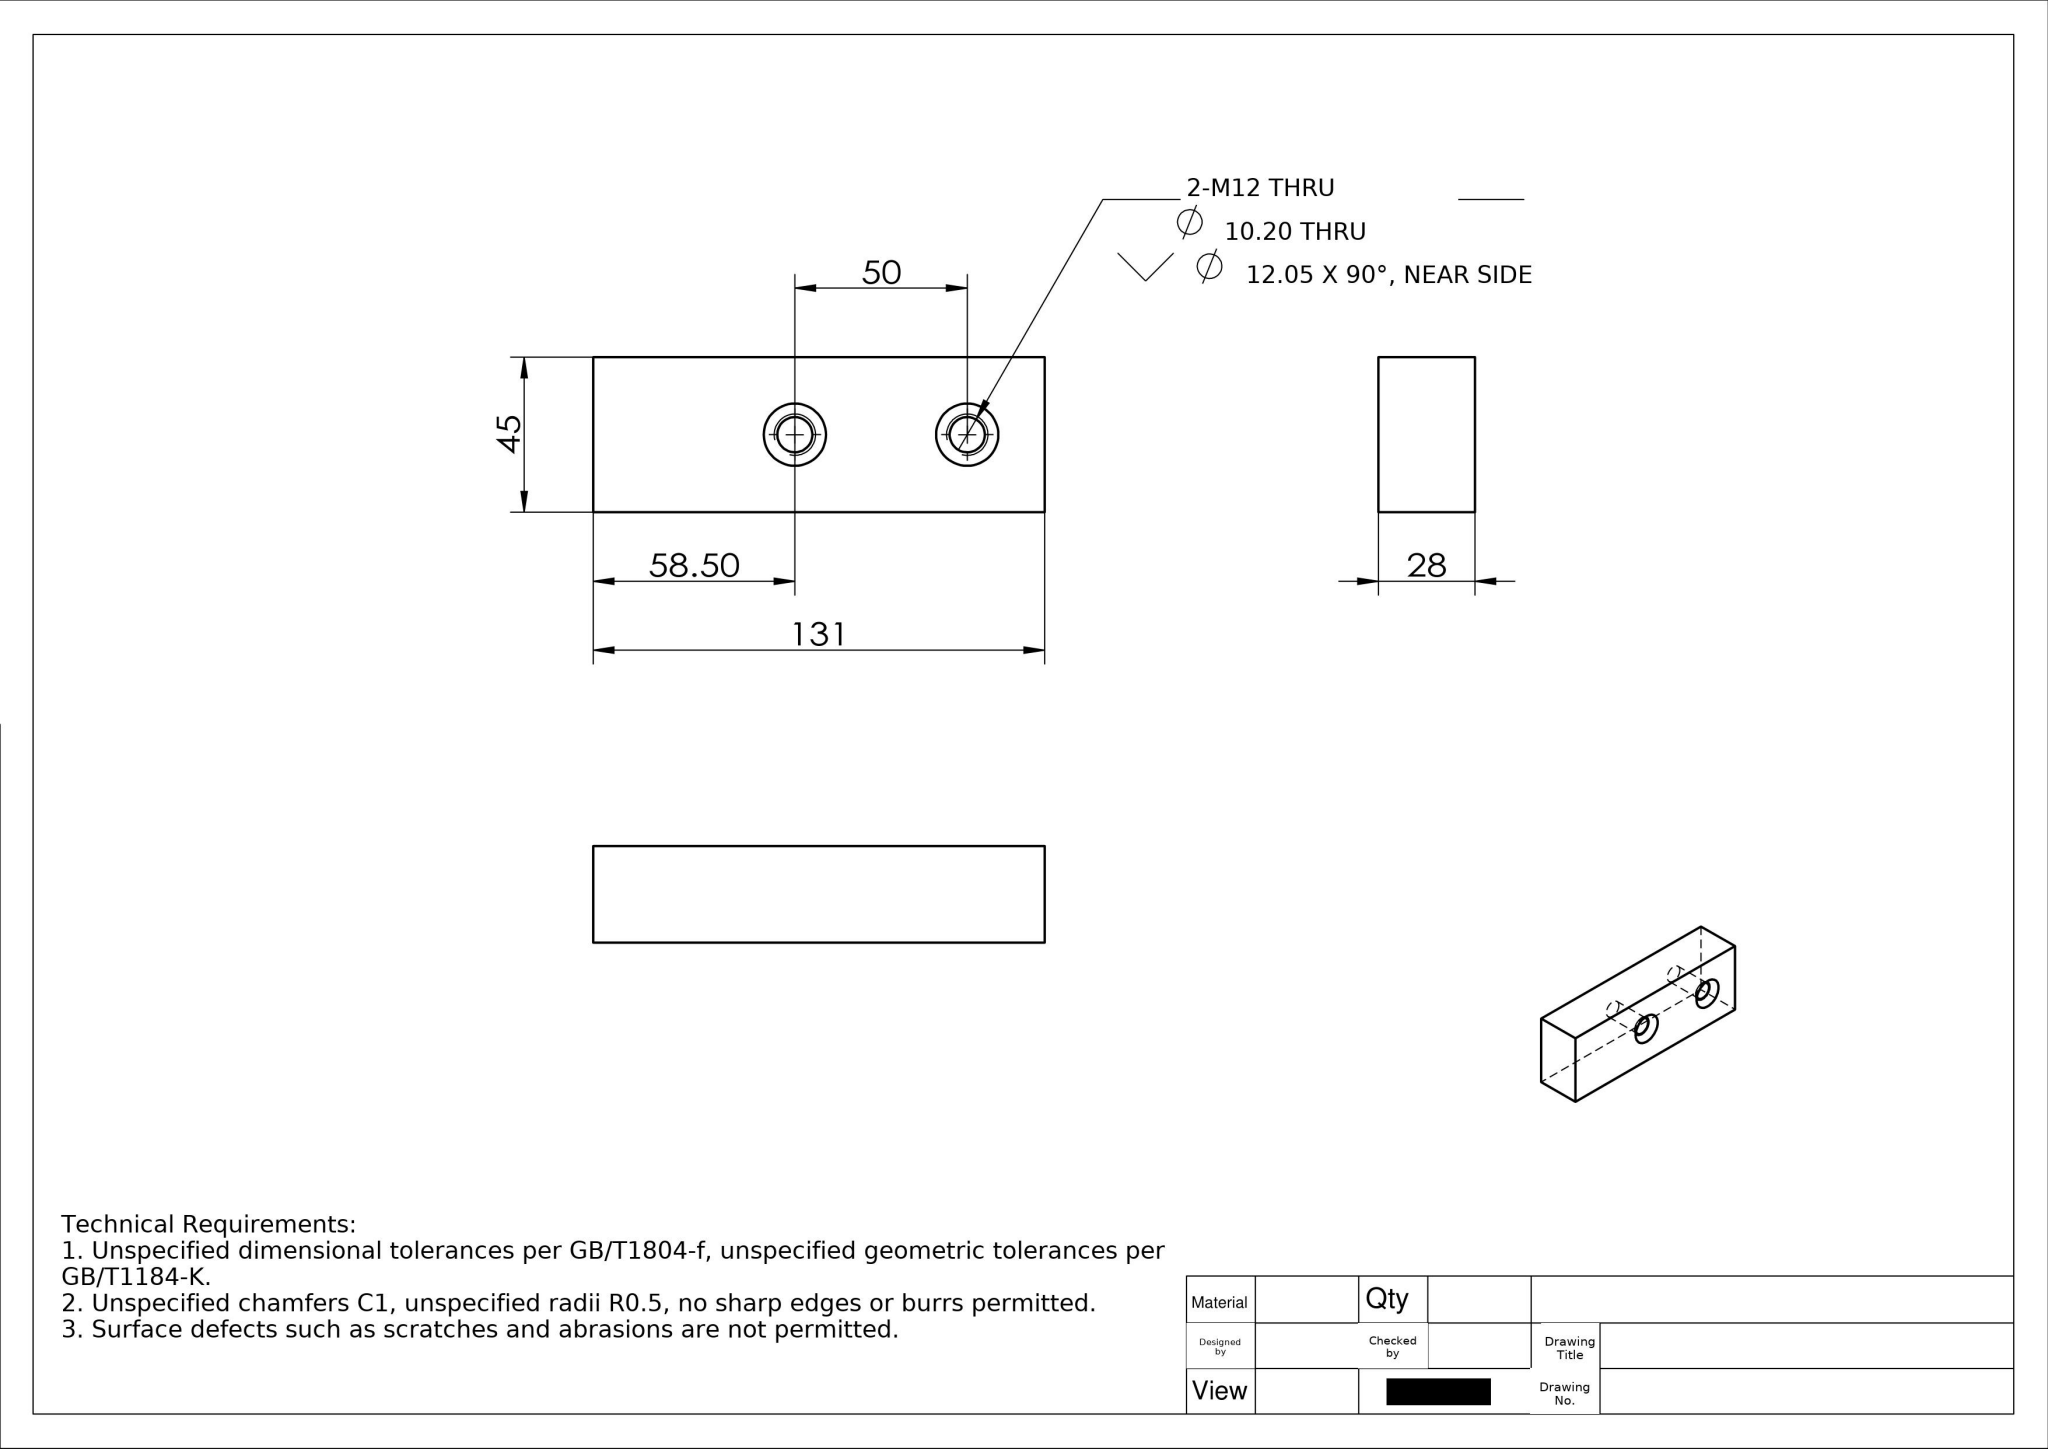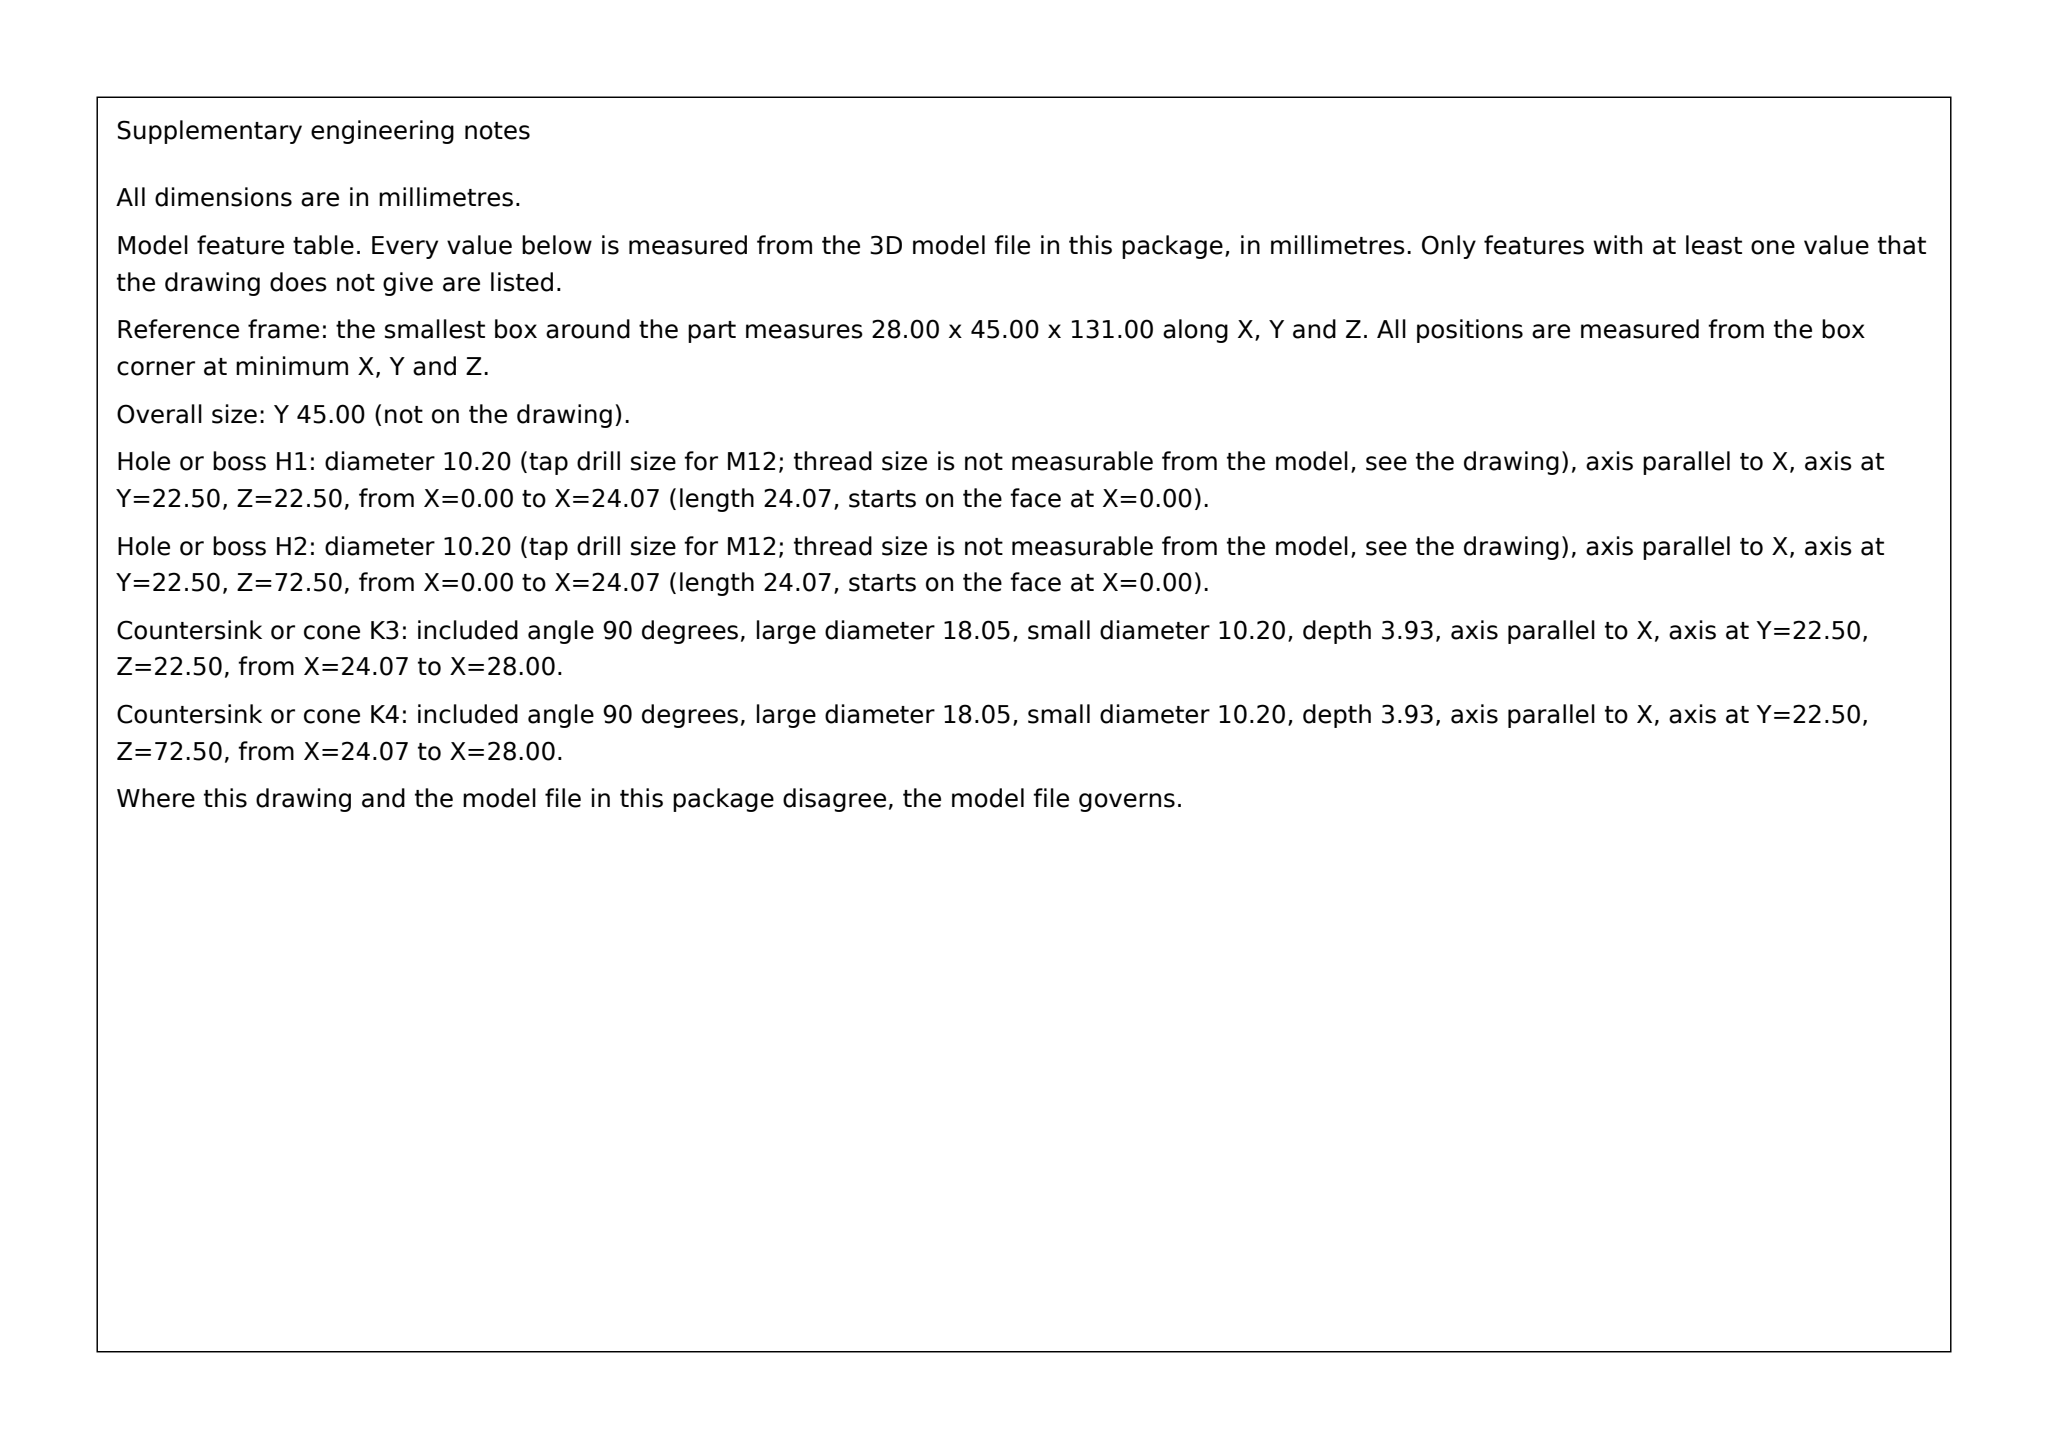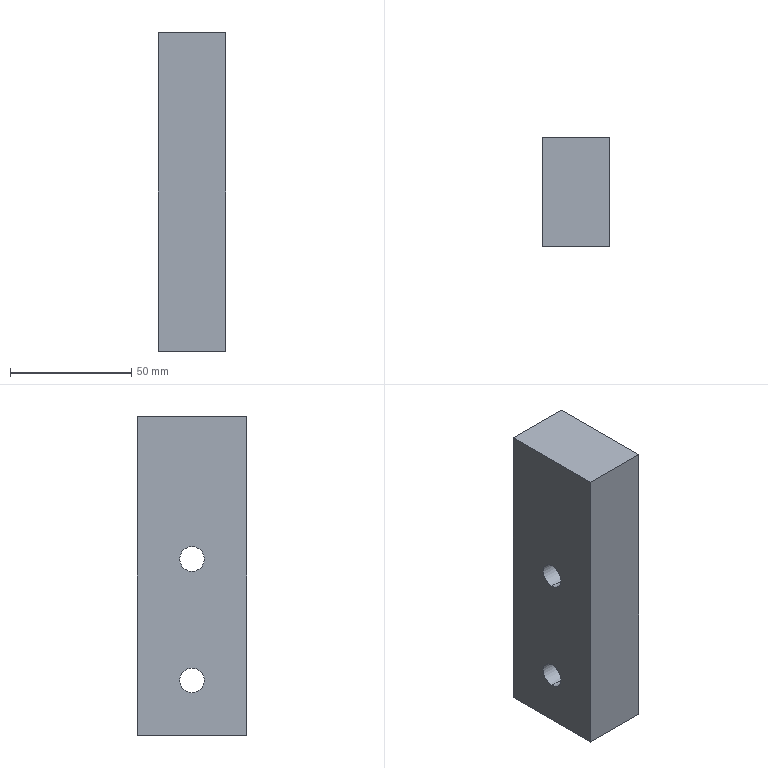Part | SolidWorks | mm | 1 solid | 14 faces | box 28 x 45 x 131 mm | volume 159864 mm3 | plane 6 | cone 4 | cylinder 4 | commonest cylinder face diameters 10.2 x4
STEP:
#1=CARTESIAN_POINT('',(-0.925,22.5,77.6));
#2=VERTEX_POINT('',#1);
#3=CARTESIAN_POINT('',(-0.925,22.5,67.4));
#4=VERTEX_POINT('',#3);
#5=CARTESIAN_POINT('',(-0.925,22.5,72.5));
#6=DIRECTION('',(1.,0.,0.));
#7=DIRECTION('',(0.,0.,-1.));
#8=AXIS2_PLACEMENT_3D('',#5,#6,#7);
#9=CIRCLE('',#8,5.1);
#10=EDGE_CURVE('',#2,#4,#9,.T.);
#11=ORIENTED_EDGE('',*,*,#10,.F.);
#12=CARTESIAN_POINT('',(3.,22.5,81.525));
#13=VERTEX_POINT('',#12);
#14=CARTESIAN_POINT('',(0.,22.5,78.525));
#15=DIRECTION('',(0.7071,0.,0.7071));
#16=VECTOR('',#15,1000.);
#17=LINE('',#14,#16);
#18=EDGE_CURVE('',#2,#13,#17,.T.);
#19=ORIENTED_EDGE('',*,*,#18,.T.);
#20=CARTESIAN_POINT('',(3.,22.5,63.475));
#21=VERTEX_POINT('',#20);
#22=CARTESIAN_POINT('',(3.,22.5,72.5));
#23=DIRECTION('',(1.,0.,0.));
#24=DIRECTION('',(0.,0.,-1.));
#25=AXIS2_PLACEMENT_3D('',#22,#23,#24);
#26=CIRCLE('',#25,9.025);
#27=EDGE_CURVE('',#13,#21,#26,.T.);
#28=ORIENTED_EDGE('',*,*,#27,.T.);
#29=CARTESIAN_POINT('',(0.,22.5,66.475));
#30=DIRECTION('',(0.7071,0.,-0.7071));
#31=VECTOR('',#30,1000.);
#32=LINE('',#29,#31);
#33=EDGE_CURVE('',#4,#21,#32,.T.);
#34=ORIENTED_EDGE('',*,*,#33,.F.);
#35=EDGE_LOOP('',(#11,#19,#28,#34));
#36=FACE_OUTER_BOUND('',#35,.T.);
#37=CARTESIAN_POINT('',(0.,22.5,72.5));
#38=DIRECTION('',(1.,0.,0.));
#39=DIRECTION('',(0.,0.,-1.));
#40=AXIS2_PLACEMENT_3D('',#37,#38,#39);
#41=CONICAL_SURFACE('',#40,6.025,0.7854);
#42=ADVANCED_FACE('',(#36),#41,.F.);
#43=CARTESIAN_POINT('',(-25.,22.5,77.6));
#44=VERTEX_POINT('',#43);
#45=CARTESIAN_POINT('',(-25.,22.5,67.4));
#46=VERTEX_POINT('',#45);
#47=CARTESIAN_POINT('',(-25.,22.5,72.5));
#48=DIRECTION('',(1.,0.,0.));
#49=DIRECTION('',(0.,0.,-1.));
#50=AXIS2_PLACEMENT_3D('',#47,#48,#49);
#51=CIRCLE('',#50,5.1);
#52=EDGE_CURVE('',#44,#46,#51,.T.);
#53=ORIENTED_EDGE('',*,*,#52,.F.);
#54=CARTESIAN_POINT('',(0.,22.5,77.6));
#55=DIRECTION('',(1.,0.,0.));
#56=VECTOR('',#55,1000.);
#57=LINE('',#54,#56);
#58=EDGE_CURVE('',#44,#2,#57,.T.);
#59=ORIENTED_EDGE('',*,*,#58,.T.);
#60=ORIENTED_EDGE('',*,*,#10,.T.);
#61=CARTESIAN_POINT('',(0.,22.5,67.4));
#62=DIRECTION('',(1.,0.,0.));
#63=VECTOR('',#62,1000.);
#64=LINE('',#61,#63);
#65=EDGE_CURVE('',#46,#4,#64,.T.);
#66=ORIENTED_EDGE('',*,*,#65,.F.);
#67=EDGE_LOOP('',(#53,#59,#60,#66));
#68=FACE_OUTER_BOUND('',#67,.T.);
#69=CARTESIAN_POINT('',(0.,22.5,72.5));
#70=DIRECTION('',(1.,0.,0.));
#71=DIRECTION('',(0.,0.,-1.));
#72=AXIS2_PLACEMENT_3D('',#69,#70,#71);
#73=CYLINDRICAL_SURFACE('',#72,5.1);
#74=ADVANCED_FACE('',(#68),#73,.F.);
#75=CARTESIAN_POINT('',(-0.925,22.5,27.6));
#76=VERTEX_POINT('',#75);
#77=CARTESIAN_POINT('',(-0.925,22.5,17.4));
#78=VERTEX_POINT('',#77);
#79=CARTESIAN_POINT('',(-0.925,22.5,22.5));
#80=DIRECTION('',(1.,0.,0.));
#81=DIRECTION('',(0.,0.,-1.));
#82=AXIS2_PLACEMENT_3D('',#79,#80,#81);
#83=CIRCLE('',#82,5.1);
#84=EDGE_CURVE('',#76,#78,#83,.T.);
#85=ORIENTED_EDGE('',*,*,#84,.F.);
#86=CARTESIAN_POINT('',(3.,22.5,31.525));
#87=VERTEX_POINT('',#86);
#88=CARTESIAN_POINT('',(0.,22.5,28.525));
#89=DIRECTION('',(0.7071,0.,0.7071));
#90=VECTOR('',#89,1000.);
#91=LINE('',#88,#90);
#92=EDGE_CURVE('',#76,#87,#91,.T.);
#93=ORIENTED_EDGE('',*,*,#92,.T.);
#94=CARTESIAN_POINT('',(3.,22.5,13.475));
#95=VERTEX_POINT('',#94);
#96=CARTESIAN_POINT('',(3.,22.5,22.5));
#97=DIRECTION('',(1.,0.,0.));
#98=DIRECTION('',(0.,0.,-1.));
#99=AXIS2_PLACEMENT_3D('',#96,#97,#98);
#100=CIRCLE('',#99,9.025);
#101=EDGE_CURVE('',#87,#95,#100,.T.);
#102=ORIENTED_EDGE('',*,*,#101,.T.);
#103=CARTESIAN_POINT('',(0.,22.5,16.475));
#104=DIRECTION('',(0.7071,0.,-0.7071));
#105=VECTOR('',#104,1000.);
#106=LINE('',#103,#105);
#107=EDGE_CURVE('',#78,#95,#106,.T.);
#108=ORIENTED_EDGE('',*,*,#107,.F.);
#109=EDGE_LOOP('',(#85,#93,#102,#108));
#110=FACE_OUTER_BOUND('',#109,.T.);
#111=CARTESIAN_POINT('',(0.,22.5,22.5));
#112=DIRECTION('',(1.,0.,0.));
#113=DIRECTION('',(0.,0.,-1.));
#114=AXIS2_PLACEMENT_3D('',#111,#112,#113);
#115=CONICAL_SURFACE('',#114,6.025,0.7854);
#116=ADVANCED_FACE('',(#110),#115,.F.);
#117=CARTESIAN_POINT('',(-25.,22.5,27.6));
#118=VERTEX_POINT('',#117);
#119=CARTESIAN_POINT('',(-25.,22.5,17.4));
#120=VERTEX_POINT('',#119);
#121=CARTESIAN_POINT('',(-25.,22.5,22.5));
#122=DIRECTION('',(1.,0.,0.));
#123=DIRECTION('',(0.,0.,-1.));
#124=AXIS2_PLACEMENT_3D('',#121,#122,#123);
#125=CIRCLE('',#124,5.1);
#126=EDGE_CURVE('',#118,#120,#125,.T.);
#127=ORIENTED_EDGE('',*,*,#126,.F.);
#128=CARTESIAN_POINT('',(0.,22.5,27.6));
#129=DIRECTION('',(1.,0.,0.));
#130=VECTOR('',#129,1000.);
#131=LINE('',#128,#130);
#132=EDGE_CURVE('',#118,#76,#131,.T.);
#133=ORIENTED_EDGE('',*,*,#132,.T.);
#134=ORIENTED_EDGE('',*,*,#84,.T.);
#135=CARTESIAN_POINT('',(0.,22.5,17.4));
#136=DIRECTION('',(1.,0.,0.));
#137=VECTOR('',#136,1000.);
#138=LINE('',#135,#137);
#139=EDGE_CURVE('',#120,#78,#138,.T.);
#140=ORIENTED_EDGE('',*,*,#139,.F.);
#141=EDGE_LOOP('',(#127,#133,#134,#140));
#142=FACE_OUTER_BOUND('',#141,.T.);
#143=CARTESIAN_POINT('',(0.,22.5,22.5));
#144=DIRECTION('',(1.,0.,0.));
#145=DIRECTION('',(0.,0.,-1.));
#146=AXIS2_PLACEMENT_3D('',#143,#144,#145);
#147=CYLINDRICAL_SURFACE('',#146,5.1);
#148=ADVANCED_FACE('',(#142),#147,.F.);
#149=CARTESIAN_POINT('',(-25.,0.,0.));
#150=VERTEX_POINT('',#149);
#151=CARTESIAN_POINT('',(-25.,0.,131.));
#152=VERTEX_POINT('',#151);
#153=CARTESIAN_POINT('',(-25.,-0.,131.));
#154=DIRECTION('',(0.,0.,1.));
#155=VECTOR('',#154,1000.);
#156=LINE('',#153,#155);
#157=EDGE_CURVE('',#150,#152,#156,.T.);
#158=ORIENTED_EDGE('',*,*,#157,.F.);
#159=CARTESIAN_POINT('',(3.,0.,0.));
#160=VERTEX_POINT('',#159);
#161=CARTESIAN_POINT('',(0.,0.,0.));
#162=DIRECTION('',(-1.,-0.,0.));
#163=VECTOR('',#162,1000.);
#164=LINE('',#161,#163);
#165=EDGE_CURVE('',#160,#150,#164,.T.);
#166=ORIENTED_EDGE('',*,*,#165,.F.);
#167=CARTESIAN_POINT('',(3.,0.,131.));
#168=VERTEX_POINT('',#167);
#169=CARTESIAN_POINT('',(3.,0.,131.));
#170=DIRECTION('',(0.,0.,-1.));
#171=VECTOR('',#170,1000.);
#172=LINE('',#169,#171);
#173=EDGE_CURVE('',#168,#160,#172,.T.);
#174=ORIENTED_EDGE('',*,*,#173,.F.);
#175=CARTESIAN_POINT('',(0.,0.,131.));
#176=DIRECTION('',(-1.,-0.,0.));
#177=VECTOR('',#176,1000.);
#178=LINE('',#175,#177);
#179=EDGE_CURVE('',#168,#152,#178,.T.);
#180=ORIENTED_EDGE('',*,*,#179,.T.);
#181=EDGE_LOOP('',(#158,#166,#174,#180));
#182=FACE_OUTER_BOUND('',#181,.T.);
#183=CARTESIAN_POINT('',(0.,0.,131.));
#184=DIRECTION('',(0.,-1.,0.));
#185=DIRECTION('',(1.,0.,0.));
#186=AXIS2_PLACEMENT_3D('',#183,#184,#185);
#187=PLANE('',#186);
#188=ADVANCED_FACE('',(#182),#187,.T.);
#189=CARTESIAN_POINT('',(3.,22.5,72.5));
#190=DIRECTION('',(1.,0.,0.));
#191=DIRECTION('',(0.,0.,-1.));
#192=AXIS2_PLACEMENT_3D('',#189,#190,#191);
#193=CIRCLE('',#192,9.025);
#194=EDGE_CURVE('',#21,#13,#193,.T.);
#195=ORIENTED_EDGE('',*,*,#194,.F.);
#196=ORIENTED_EDGE('',*,*,#27,.F.);
#197=EDGE_LOOP('',(#195,#196));
#198=FACE_BOUND('',#197,.T.);
#199=CARTESIAN_POINT('',(3.,22.5,22.5));
#200=DIRECTION('',(1.,0.,0.));
#201=DIRECTION('',(0.,0.,-1.));
#202=AXIS2_PLACEMENT_3D('',#199,#200,#201);
#203=CIRCLE('',#202,9.025);
#204=EDGE_CURVE('',#95,#87,#203,.T.);
#205=ORIENTED_EDGE('',*,*,#204,.F.);
#206=ORIENTED_EDGE('',*,*,#101,.F.);
#207=EDGE_LOOP('',(#205,#206));
#208=FACE_BOUND('',#207,.T.);
#209=CARTESIAN_POINT('',(3.,45.,0.));
#210=VERTEX_POINT('',#209);
#211=CARTESIAN_POINT('',(3.,0.,0.));
#212=DIRECTION('',(0.,-1.,0.));
#213=VECTOR('',#212,1000.);
#214=LINE('',#211,#213);
#215=EDGE_CURVE('',#210,#160,#214,.T.);
#216=ORIENTED_EDGE('',*,*,#215,.F.);
#217=CARTESIAN_POINT('',(3.,45.,131.));
#218=VERTEX_POINT('',#217);
#219=CARTESIAN_POINT('',(3.,45.,131.));
#220=DIRECTION('',(0.,0.,-1.));
#221=VECTOR('',#220,1000.);
#222=LINE('',#219,#221);
#223=EDGE_CURVE('',#218,#210,#222,.T.);
#224=ORIENTED_EDGE('',*,*,#223,.F.);
#225=CARTESIAN_POINT('',(3.,0.,131.));
#226=DIRECTION('',(0.,-1.,0.));
#227=VECTOR('',#226,1000.);
#228=LINE('',#225,#227);
#229=EDGE_CURVE('',#218,#168,#228,.T.);
#230=ORIENTED_EDGE('',*,*,#229,.T.);
#231=ORIENTED_EDGE('',*,*,#173,.T.);
#232=EDGE_LOOP('',(#216,#224,#230,#231));
#233=FACE_OUTER_BOUND('',#232,.T.);
#234=CARTESIAN_POINT('',(3.,0.,131.));
#235=DIRECTION('',(1.,0.,0.));
#236=DIRECTION('',(0.,0.,-1.));
#237=AXIS2_PLACEMENT_3D('',#234,#235,#236);
#238=PLANE('',#237);
#239=ADVANCED_FACE('',(#198,#208,#233),#238,.T.);
#240=CARTESIAN_POINT('',(-25.,45.,0.));
#241=VERTEX_POINT('',#240);
#242=CARTESIAN_POINT('',(-25.,45.,0.));
#243=DIRECTION('',(1.,0.,0.));
#244=VECTOR('',#243,1000.);
#245=LINE('',#242,#244);
#246=EDGE_CURVE('',#241,#210,#245,.T.);
#247=ORIENTED_EDGE('',*,*,#246,.F.);
#248=CARTESIAN_POINT('',(-25.,45.,131.));
#249=VERTEX_POINT('',#248);
#250=CARTESIAN_POINT('',(-25.,45.,131.));
#251=DIRECTION('',(0.,0.,-1.));
#252=VECTOR('',#251,1000.);
#253=LINE('',#250,#252);
#254=EDGE_CURVE('',#249,#241,#253,.T.);
#255=ORIENTED_EDGE('',*,*,#254,.F.);
#256=CARTESIAN_POINT('',(-25.,45.,131.));
#257=DIRECTION('',(1.,0.,0.));
#258=VECTOR('',#257,1000.);
#259=LINE('',#256,#258);
#260=EDGE_CURVE('',#249,#218,#259,.T.);
#261=ORIENTED_EDGE('',*,*,#260,.T.);
#262=ORIENTED_EDGE('',*,*,#223,.T.);
#263=EDGE_LOOP('',(#247,#255,#261,#262));
#264=FACE_OUTER_BOUND('',#263,.T.);
#265=CARTESIAN_POINT('',(-25.,45.,131.));
#266=DIRECTION('',(-0.,1.,0.));
#267=DIRECTION('',(-1.,-0.,0.));
#268=AXIS2_PLACEMENT_3D('',#265,#266,#267);
#269=PLANE('',#268);
#270=ADVANCED_FACE('',(#264),#269,.T.);
#271=CARTESIAN_POINT('',(-25.,0.,0.));
#272=DIRECTION('',(0.,-1.,0.));
#273=VECTOR('',#272,1000.);
#274=LINE('',#271,#273);
#275=EDGE_CURVE('',#241,#150,#274,.T.);
#276=ORIENTED_EDGE('',*,*,#275,.T.);
#277=ORIENTED_EDGE('',*,*,#157,.T.);
#278=CARTESIAN_POINT('',(-25.,0.,131.));
#279=DIRECTION('',(0.,-1.,0.));
#280=VECTOR('',#279,1000.);
#281=LINE('',#278,#280);
#282=EDGE_CURVE('',#249,#152,#281,.T.);
#283=ORIENTED_EDGE('',*,*,#282,.F.);
#284=ORIENTED_EDGE('',*,*,#254,.T.);
#285=EDGE_LOOP('',(#276,#277,#283,#284));
#286=FACE_OUTER_BOUND('',#285,.T.);
#287=CARTESIAN_POINT('',(-25.,22.5,22.5));
#288=DIRECTION('',(1.,0.,0.));
#289=DIRECTION('',(0.,0.,-1.));
#290=AXIS2_PLACEMENT_3D('',#287,#288,#289);
#291=CIRCLE('',#290,5.1);
#292=EDGE_CURVE('',#120,#118,#291,.T.);
#293=ORIENTED_EDGE('',*,*,#292,.T.);
#294=ORIENTED_EDGE('',*,*,#126,.T.);
#295=EDGE_LOOP('',(#293,#294));
#296=FACE_BOUND('',#295,.T.);
#297=CARTESIAN_POINT('',(-25.,22.5,72.5));
#298=DIRECTION('',(1.,0.,0.));
#299=DIRECTION('',(0.,0.,-1.));
#300=AXIS2_PLACEMENT_3D('',#297,#298,#299);
#301=CIRCLE('',#300,5.1);
#302=EDGE_CURVE('',#46,#44,#301,.T.);
#303=ORIENTED_EDGE('',*,*,#302,.T.);
#304=ORIENTED_EDGE('',*,*,#52,.T.);
#305=EDGE_LOOP('',(#303,#304));
#306=FACE_BOUND('',#305,.T.);
#307=CARTESIAN_POINT('',(-25.,0.,131.));
#308=DIRECTION('',(1.,0.,0.));
#309=DIRECTION('',(0.,0.,-1.));
#310=AXIS2_PLACEMENT_3D('',#307,#308,#309);
#311=PLANE('',#310);
#312=ADVANCED_FACE('',(#286,#296,#306),#311,.F.);
#313=ORIENTED_EDGE('',*,*,#282,.T.);
#314=ORIENTED_EDGE('',*,*,#179,.F.);
#315=ORIENTED_EDGE('',*,*,#229,.F.);
#316=ORIENTED_EDGE('',*,*,#260,.F.);
#317=EDGE_LOOP('',(#313,#314,#315,#316));
#318=FACE_OUTER_BOUND('',#317,.T.);
#319=CARTESIAN_POINT('',(0.,0.,131.));
#320=DIRECTION('',(0.,0.,-1.));
#321=DIRECTION('',(-1.,0.,0.));
#322=AXIS2_PLACEMENT_3D('',#319,#320,#321);
#323=PLANE('',#322);
#324=ADVANCED_FACE('',(#318),#323,.F.);
#325=ORIENTED_EDGE('',*,*,#165,.T.);
#326=ORIENTED_EDGE('',*,*,#275,.F.);
#327=ORIENTED_EDGE('',*,*,#246,.T.);
#328=ORIENTED_EDGE('',*,*,#215,.T.);
#329=EDGE_LOOP('',(#325,#326,#327,#328));
#330=FACE_OUTER_BOUND('',#329,.T.);
#331=CARTESIAN_POINT('',(0.,0.,0.));
#332=DIRECTION('',(0.,0.,-1.));
#333=DIRECTION('',(-1.,0.,0.));
#334=AXIS2_PLACEMENT_3D('',#331,#332,#333);
#335=PLANE('',#334);
#336=ADVANCED_FACE('',(#330),#335,.T.);
#337=ORIENTED_EDGE('',*,*,#132,.F.);
#338=ORIENTED_EDGE('',*,*,#292,.F.);
#339=ORIENTED_EDGE('',*,*,#139,.T.);
#340=CARTESIAN_POINT('',(-0.925,22.5,22.5));
#341=DIRECTION('',(1.,0.,0.));
#342=DIRECTION('',(0.,0.,-1.));
#343=AXIS2_PLACEMENT_3D('',#340,#341,#342);
#344=CIRCLE('',#343,5.1);
#345=EDGE_CURVE('',#78,#76,#344,.T.);
#346=ORIENTED_EDGE('',*,*,#345,.T.);
#347=EDGE_LOOP('',(#337,#338,#339,#346));
#348=FACE_OUTER_BOUND('',#347,.T.);
#349=CARTESIAN_POINT('',(0.,22.5,22.5));
#350=DIRECTION('',(1.,0.,0.));
#351=DIRECTION('',(0.,0.,-1.));
#352=AXIS2_PLACEMENT_3D('',#349,#350,#351);
#353=CYLINDRICAL_SURFACE('',#352,5.1);
#354=ADVANCED_FACE('',(#348),#353,.F.);
#355=ORIENTED_EDGE('',*,*,#92,.F.);
#356=ORIENTED_EDGE('',*,*,#345,.F.);
#357=ORIENTED_EDGE('',*,*,#107,.T.);
#358=ORIENTED_EDGE('',*,*,#204,.T.);
#359=EDGE_LOOP('',(#355,#356,#357,#358));
#360=FACE_OUTER_BOUND('',#359,.T.);
#361=CARTESIAN_POINT('',(0.,22.5,22.5));
#362=DIRECTION('',(1.,0.,0.));
#363=DIRECTION('',(0.,0.,-1.));
#364=AXIS2_PLACEMENT_3D('',#361,#362,#363);
#365=CONICAL_SURFACE('',#364,6.025,0.7854);
#366=ADVANCED_FACE('',(#360),#365,.F.);
#367=ORIENTED_EDGE('',*,*,#58,.F.);
#368=ORIENTED_EDGE('',*,*,#302,.F.);
#369=ORIENTED_EDGE('',*,*,#65,.T.);
#370=CARTESIAN_POINT('',(-0.925,22.5,72.5));
#371=DIRECTION('',(1.,0.,0.));
#372=DIRECTION('',(0.,0.,-1.));
#373=AXIS2_PLACEMENT_3D('',#370,#371,#372);
#374=CIRCLE('',#373,5.1);
#375=EDGE_CURVE('',#4,#2,#374,.T.);
#376=ORIENTED_EDGE('',*,*,#375,.T.);
#377=EDGE_LOOP('',(#367,#368,#369,#376));
#378=FACE_OUTER_BOUND('',#377,.T.);
#379=CARTESIAN_POINT('',(0.,22.5,72.5));
#380=DIRECTION('',(1.,0.,0.));
#381=DIRECTION('',(0.,0.,-1.));
#382=AXIS2_PLACEMENT_3D('',#379,#380,#381);
#383=CYLINDRICAL_SURFACE('',#382,5.1);
#384=ADVANCED_FACE('',(#378),#383,.F.);
#385=ORIENTED_EDGE('',*,*,#18,.F.);
#386=ORIENTED_EDGE('',*,*,#375,.F.);
#387=ORIENTED_EDGE('',*,*,#33,.T.);
#388=ORIENTED_EDGE('',*,*,#194,.T.);
#389=EDGE_LOOP('',(#385,#386,#387,#388));
#390=FACE_OUTER_BOUND('',#389,.T.);
#391=CARTESIAN_POINT('',(0.,22.5,72.5));
#392=DIRECTION('',(1.,0.,0.));
#393=DIRECTION('',(0.,0.,-1.));
#394=AXIS2_PLACEMENT_3D('',#391,#392,#393);
#395=CONICAL_SURFACE('',#394,6.025,0.7854);
#396=ADVANCED_FACE('',(#390),#395,.F.);
#397=CLOSED_SHELL('',(#42,#74,#116,#148,#188,#239,#270,#312,#324,#336,#354,#366,#384,#396));
#398=MANIFOLD_SOLID_BREP('',#397);
#399=CARTESIAN_POINT('',(0.,0.,0.));
#400=DIRECTION('',(0.,0.,1.));
#401=DIRECTION('',(1.,0.,0.));
#402=AXIS2_PLACEMENT_3D('',#399,#400,#401);
#403=(LENGTH_UNIT()NAMED_UNIT(*)SI_UNIT(.MILLI.,.METRE.));
#404=UNCERTAINTY_MEASURE_WITH_UNIT(LENGTH_MEASURE(0.00001),#403,'','');
#405=(NAMED_UNIT(*)PLANE_ANGLE_UNIT()SI_UNIT($,.RADIAN.));
#406=(NAMED_UNIT(*)SI_UNIT($,.STERADIAN.)SOLID_ANGLE_UNIT());
#407=(GEOMETRIC_REPRESENTATION_CONTEXT(3)GLOBAL_UNCERTAINTY_ASSIGNED_CONTEXT((#404))GLOBAL_UNIT_ASSIGNED_CONTEXT((#403,#405,#406))REPRESENTATION_CONTEXT('',''));
#408=ADVANCED_BREP_SHAPE_REPRESENTATION('',(#398,#402),#407);